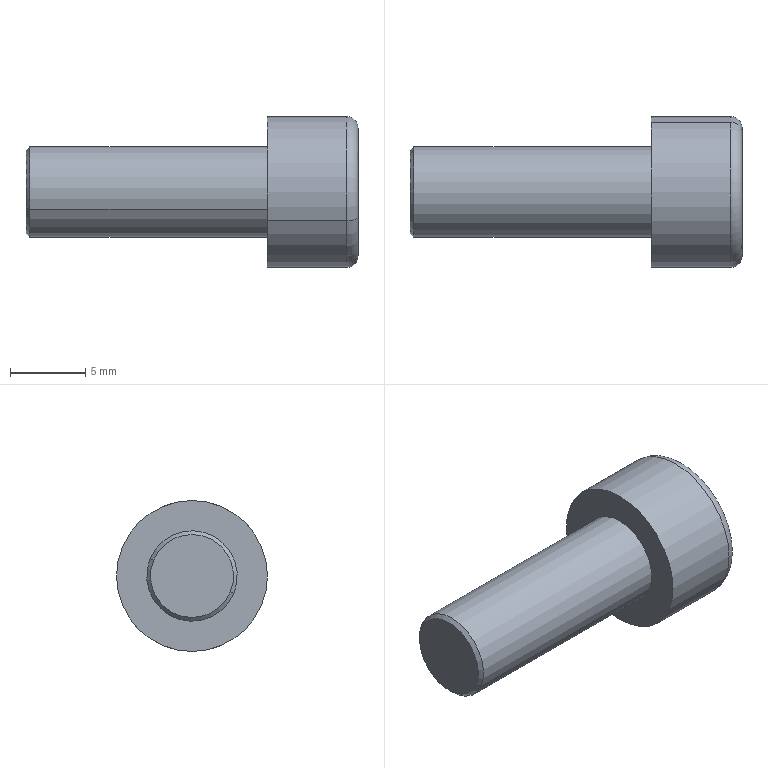Component | SolidWorks | hexagon socket head cap screws gb-11 | 1 solid | 25 faces | volume 845 mm3 | plane 15 | cone 4 | cylinder 4 | torus 2 | commonest cylinder face diameters 6 x2 10 x2